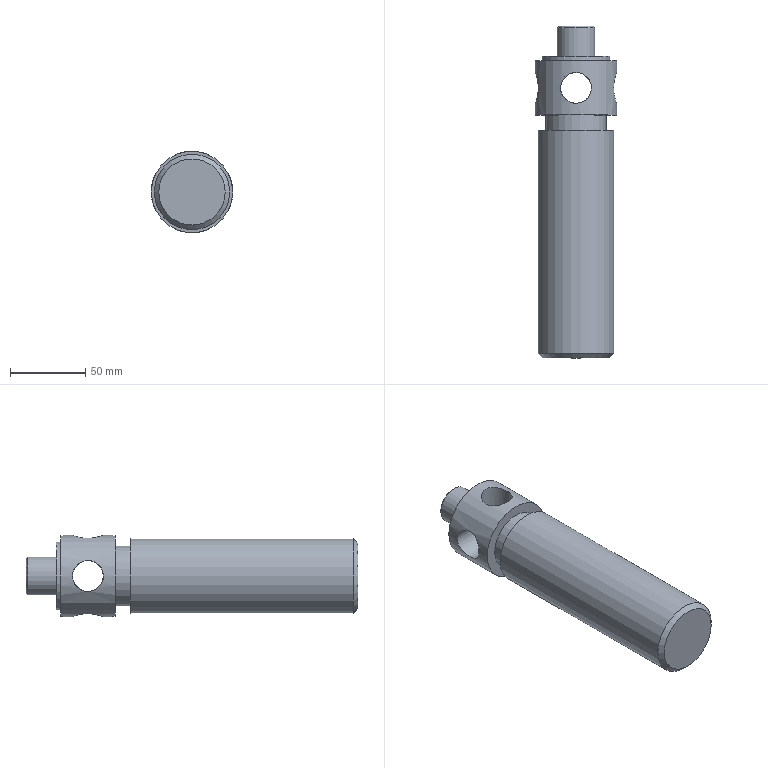Component | NX | LEAD_SCREW | 1 solid | 20 faces | volume 374947 mm3 | cylinder 10 | plane 6 | cone 4 | commonest cylinder face diameters 20.5 x4 54 x1 50 x1 25 x1 45 x1 40 x1 8.5 x1